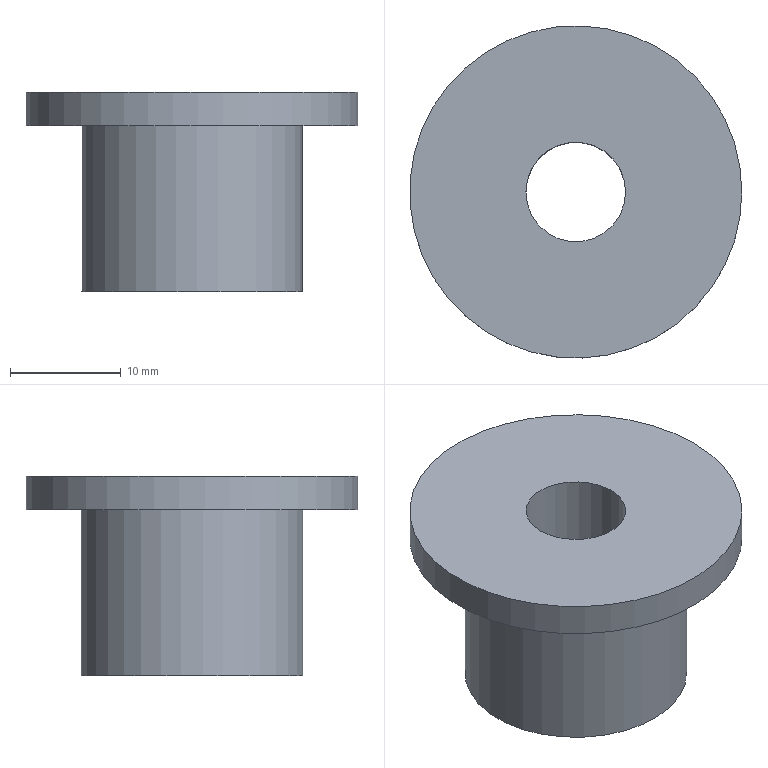Component | NX | ROLLING_SHAFT | 1 solid | 6 faces | box 30 x 30 x 18 mm | volume 5688 mm3 | cylinder 3 | plane 3 | commonest cylinder face diameters 30 x1 9 x1 20 x1
STEP:
#1=CARTESIAN_POINT('',(0.,0.,0.));
#2=DIRECTION('',(0.,0.,1.));
#3=DIRECTION('',(1.,0.,0.));
#4=AXIS2_PLACEMENT_3D('',#1,#2,#3);
#5=CARTESIAN_POINT('',(1475.132,1212.,819.574));
#6=VERTEX_POINT('',#5);
#7=CARTESIAN_POINT('',(1460.132,1212.,819.574));
#8=DIRECTION('',(0.,0.,1.));
#9=DIRECTION('',(1.,0.,0.));
#10=AXIS2_PLACEMENT_3D('',#7,#8,#9);
#11=CIRCLE('',#10,15.);
#12=CARTESIAN_POINT('',(1460.132,1212.,819.574));
#13=DIRECTION('',(0.,0.,1.));
#14=DIRECTION('',(1.,0.,0.));
#15=AXIS2_PLACEMENT_3D('',#12,#13,#14);
#16=CYLINDRICAL_SURFACE('',#15,15.);
#17=CARTESIAN_POINT('',(0.,0.));
#18=DIRECTION('',(1.,0.));
#19=VECTOR('',#18,1.);
#20=LINE('',#17,#19);
#21=(GEOMETRIC_REPRESENTATION_CONTEXT(2)PARAMETRIC_REPRESENTATION_CONTEXT()REPRESENTATION_CONTEXT('',''));
#22=DEFINITIONAL_REPRESENTATION('',(#20),#21);
#23=PCURVE('',#16,#22);
#24=CARTESIAN_POINT('',(1460.132,1212.,819.574));
#25=DIRECTION('',(0.,0.,1.));
#26=DIRECTION('',(1.,0.,0.));
#27=AXIS2_PLACEMENT_3D('',#24,#25,#26);
#28=PLANE('',#27);
#29=CARTESIAN_POINT('',(0.,0.));
#30=DIRECTION('',(1.,0.));
#31=AXIS2_PLACEMENT_2D('',#29,#30);
#32=CIRCLE('',#31,15.);
#33=(GEOMETRIC_REPRESENTATION_CONTEXT(2)PARAMETRIC_REPRESENTATION_CONTEXT()REPRESENTATION_CONTEXT('',''));
#34=DEFINITIONAL_REPRESENTATION('',(#32),#33);
#35=PCURVE('',#28,#34);
#36=SURFACE_CURVE('',#11,(#23,#35),.PCURVE_S1.);
#37=EDGE_CURVE('',#6,#6,#36,.T.);
#38=ORIENTED_EDGE('',*,*,#37,.T.);
#39=CARTESIAN_POINT('',(1475.132,1212.,822.574));
#40=VERTEX_POINT('',#39);
#41=CARTESIAN_POINT('',(1475.132,1212.,819.574));
#42=CARTESIAN_POINT('',(1475.132,1212.,822.574));
#43=B_SPLINE_CURVE_WITH_KNOTS('',1,(#41,#42),.UNSPECIFIED.,.F.,.F.,(2,2),(0.,3.),.PIECEWISE_BEZIER_KNOTS.);
#44=CARTESIAN_POINT('',(6.283,0.));
#45=DIRECTION('',(0.,1.));
#46=VECTOR('',#45,1.);
#47=LINE('',#44,#46);
#48=(GEOMETRIC_REPRESENTATION_CONTEXT(2)PARAMETRIC_REPRESENTATION_CONTEXT()REPRESENTATION_CONTEXT('',''));
#49=DEFINITIONAL_REPRESENTATION('',(#47),#48);
#50=PCURVE('',#16,#49);
#51=CARTESIAN_POINT('',(0.,0.));
#52=DIRECTION('',(0.,1.));
#53=VECTOR('',#52,1.);
#54=LINE('',#51,#53);
#55=(GEOMETRIC_REPRESENTATION_CONTEXT(2)PARAMETRIC_REPRESENTATION_CONTEXT()REPRESENTATION_CONTEXT('',''));
#56=DEFINITIONAL_REPRESENTATION('',(#54),#55);
#57=PCURVE('',#16,#56);
#58=SEAM_CURVE('',#43,(#50,#57),.PCURVE_S1.);
#59=EDGE_CURVE('',#6,#40,#58,.T.);
#60=ORIENTED_EDGE('',*,*,#59,.T.);
#61=CARTESIAN_POINT('',(1460.132,1212.,822.574));
#62=DIRECTION('',(0.,0.,1.));
#63=DIRECTION('',(1.,0.,0.));
#64=AXIS2_PLACEMENT_3D('',#61,#62,#63);
#65=CIRCLE('',#64,15.);
#66=CARTESIAN_POINT('',(0.,3.));
#67=DIRECTION('',(1.,0.));
#68=VECTOR('',#67,1.);
#69=LINE('',#66,#68);
#70=(GEOMETRIC_REPRESENTATION_CONTEXT(2)PARAMETRIC_REPRESENTATION_CONTEXT()REPRESENTATION_CONTEXT('',''));
#71=DEFINITIONAL_REPRESENTATION('',(#69),#70);
#72=PCURVE('',#16,#71);
#73=CARTESIAN_POINT('',(1460.132,1212.,822.574));
#74=DIRECTION('',(0.,0.,1.));
#75=DIRECTION('',(1.,0.,0.));
#76=AXIS2_PLACEMENT_3D('',#73,#74,#75);
#77=PLANE('',#76);
#78=CARTESIAN_POINT('',(0.,0.));
#79=DIRECTION('',(1.,0.));
#80=AXIS2_PLACEMENT_2D('',#78,#79);
#81=CIRCLE('',#80,15.);
#82=(GEOMETRIC_REPRESENTATION_CONTEXT(2)PARAMETRIC_REPRESENTATION_CONTEXT()REPRESENTATION_CONTEXT('',''));
#83=DEFINITIONAL_REPRESENTATION('',(#81),#82);
#84=PCURVE('',#77,#83);
#85=SURFACE_CURVE('',#65,(#72,#84),.PCURVE_S1.);
#86=EDGE_CURVE('',#40,#40,#85,.T.);
#87=ORIENTED_EDGE('',*,*,#86,.F.);
#88=ORIENTED_EDGE('',*,*,#59,.F.);
#89=EDGE_LOOP('',(#38,#60,#87,#88));
#90=FACE_BOUND('',#89,.T.);
#91=ADVANCED_FACE('',(#90),#16,.T.);
#92=CARTESIAN_POINT('',(1464.632,1212.,822.574));
#93=VERTEX_POINT('',#92);
#94=CARTESIAN_POINT('',(1460.132,1212.,822.574));
#95=DIRECTION('',(0.,0.,1.));
#96=DIRECTION('',(1.,0.,0.));
#97=AXIS2_PLACEMENT_3D('',#94,#95,#96);
#98=CIRCLE('',#97,4.5);
#99=CARTESIAN_POINT('',(1460.132,1212.,819.574));
#100=DIRECTION('',(0.,0.,1.));
#101=DIRECTION('',(1.,0.,0.));
#102=AXIS2_PLACEMENT_3D('',#99,#100,#101);
#103=CYLINDRICAL_SURFACE('',#102,4.5);
#104=CARTESIAN_POINT('',(0.,3.));
#105=DIRECTION('',(1.,0.));
#106=VECTOR('',#105,1.);
#107=LINE('',#104,#106);
#108=(GEOMETRIC_REPRESENTATION_CONTEXT(2)PARAMETRIC_REPRESENTATION_CONTEXT()REPRESENTATION_CONTEXT('',''));
#109=DEFINITIONAL_REPRESENTATION('',(#107),#108);
#110=PCURVE('',#103,#109);
#111=CARTESIAN_POINT('',(0.,0.));
#112=DIRECTION('',(1.,0.));
#113=AXIS2_PLACEMENT_2D('',#111,#112);
#114=CIRCLE('',#113,4.5);
#115=(GEOMETRIC_REPRESENTATION_CONTEXT(2)PARAMETRIC_REPRESENTATION_CONTEXT()REPRESENTATION_CONTEXT('',''));
#116=DEFINITIONAL_REPRESENTATION('',(#114),#115);
#117=PCURVE('',#77,#116);
#118=SURFACE_CURVE('',#98,(#110,#117),.PCURVE_S1.);
#119=EDGE_CURVE('',#93,#93,#118,.T.);
#120=ORIENTED_EDGE('',*,*,#119,.F.);
#121=CARTESIAN_POINT('',(1464.632,1212.,804.574));
#122=VERTEX_POINT('',#121);
#123=CARTESIAN_POINT('',(1464.632,1212.,804.574));
#124=CARTESIAN_POINT('',(1464.632,1212.,822.574));
#125=B_SPLINE_CURVE_WITH_KNOTS('',1,(#123,#124),.UNSPECIFIED.,.F.,.F.,(2,2),(-15.,3.),.PIECEWISE_BEZIER_KNOTS.);
#126=CARTESIAN_POINT('',(0.,0.));
#127=DIRECTION('',(0.,1.));
#128=VECTOR('',#127,1.);
#129=LINE('',#126,#128);
#130=(GEOMETRIC_REPRESENTATION_CONTEXT(2)PARAMETRIC_REPRESENTATION_CONTEXT()REPRESENTATION_CONTEXT('',''));
#131=DEFINITIONAL_REPRESENTATION('',(#129),#130);
#132=PCURVE('',#103,#131);
#133=CARTESIAN_POINT('',(6.283,0.));
#134=DIRECTION('',(0.,1.));
#135=VECTOR('',#134,1.);
#136=LINE('',#133,#135);
#137=(GEOMETRIC_REPRESENTATION_CONTEXT(2)PARAMETRIC_REPRESENTATION_CONTEXT()REPRESENTATION_CONTEXT('',''));
#138=DEFINITIONAL_REPRESENTATION('',(#136),#137);
#139=PCURVE('',#103,#138);
#140=SEAM_CURVE('',#125,(#132,#139),.PCURVE_S1.);
#141=EDGE_CURVE('',#122,#93,#140,.T.);
#142=ORIENTED_EDGE('',*,*,#141,.F.);
#143=CARTESIAN_POINT('',(1460.132,1212.,804.574));
#144=DIRECTION('',(0.,0.,-1.));
#145=DIRECTION('',(1.,0.,0.));
#146=AXIS2_PLACEMENT_3D('',#143,#144,#145);
#147=CIRCLE('',#146,4.5);
#148=CARTESIAN_POINT('',(6.283,-15.));
#149=DIRECTION('',(-1.,0.));
#150=VECTOR('',#149,1.);
#151=LINE('',#148,#150);
#152=(GEOMETRIC_REPRESENTATION_CONTEXT(2)PARAMETRIC_REPRESENTATION_CONTEXT()REPRESENTATION_CONTEXT('',''));
#153=DEFINITIONAL_REPRESENTATION('',(#151),#152);
#154=PCURVE('',#103,#153);
#155=CARTESIAN_POINT('',(1460.132,1212.,804.574));
#156=DIRECTION('',(0.,0.,-1.));
#157=DIRECTION('',(-1.,0.,0.));
#158=AXIS2_PLACEMENT_3D('',#155,#156,#157);
#159=PLANE('',#158);
#160=CARTESIAN_POINT('',(0.,0.));
#161=DIRECTION('',(-1.,0.));
#162=AXIS2_PLACEMENT_2D('',#160,#161);
#163=CIRCLE('',#162,4.5);
#164=(GEOMETRIC_REPRESENTATION_CONTEXT(2)PARAMETRIC_REPRESENTATION_CONTEXT()REPRESENTATION_CONTEXT('',''));
#165=DEFINITIONAL_REPRESENTATION('',(#163),#164);
#166=PCURVE('',#159,#165);
#167=SURFACE_CURVE('',#147,(#154,#166),.PCURVE_S1.);
#168=EDGE_CURVE('',#122,#122,#167,.T.);
#169=ORIENTED_EDGE('',*,*,#168,.F.);
#170=ORIENTED_EDGE('',*,*,#141,.T.);
#171=EDGE_LOOP('',(#120,#142,#169,#170));
#172=FACE_BOUND('',#171,.F.);
#173=ADVANCED_FACE('',(#172),#103,.F.);
#174=CARTESIAN_POINT('',(1470.132,1212.,819.574));
#175=VERTEX_POINT('',#174);
#176=CARTESIAN_POINT('',(1460.132,1212.,819.574));
#177=DIRECTION('',(0.,0.,-1.));
#178=DIRECTION('',(1.,0.,0.));
#179=AXIS2_PLACEMENT_3D('',#176,#177,#178);
#180=CIRCLE('',#179,10.);
#181=CARTESIAN_POINT('',(10.,0.));
#182=CARTESIAN_POINT('',(10.,-17.321));
#183=CARTESIAN_POINT('',(-5.,-8.66));
#184=CARTESIAN_POINT('',(-20.,-0.));
#185=CARTESIAN_POINT('',(-5.,8.66));
#186=CARTESIAN_POINT('',(10.,17.321));
#187=CARTESIAN_POINT('',(10.,0.));
#188=(BOUNDED_CURVE()B_SPLINE_CURVE(2,(#181,#182,#183,#184,#185,#186,#187),.UNSPECIFIED.,.T.,.F.)B_SPLINE_CURVE_WITH_KNOTS((1,2,2,2,2,1),(-2.094,0.,2.094,4.189,6.283,8.378),.UNSPECIFIED.)CURVE()GEOMETRIC_REPRESENTATION_ITEM()RATIONAL_B_SPLINE_CURVE((1.,0.5,1.,0.5,1.,0.5,1.))REPRESENTATION_ITEM(''));
#189=(GEOMETRIC_REPRESENTATION_CONTEXT(2)PARAMETRIC_REPRESENTATION_CONTEXT()REPRESENTATION_CONTEXT('',''));
#190=DEFINITIONAL_REPRESENTATION('',(#188),#189);
#191=PCURVE('',#28,#190);
#192=CARTESIAN_POINT('',(1460.132,1212.,804.574));
#193=DIRECTION('',(0.,0.,1.));
#194=DIRECTION('',(1.,0.,0.));
#195=AXIS2_PLACEMENT_3D('',#192,#193,#194);
#196=CYLINDRICAL_SURFACE('',#195,10.);
#197=CARTESIAN_POINT('',(6.283,15.));
#198=DIRECTION('',(-1.,0.));
#199=VECTOR('',#198,1.);
#200=LINE('',#197,#199);
#201=(GEOMETRIC_REPRESENTATION_CONTEXT(2)PARAMETRIC_REPRESENTATION_CONTEXT()REPRESENTATION_CONTEXT('',''));
#202=DEFINITIONAL_REPRESENTATION('',(#200),#201);
#203=PCURVE('',#196,#202);
#204=SURFACE_CURVE('',#180,(#191,#203),.PCURVE_S1.);
#205=EDGE_CURVE('',#175,#175,#204,.T.);
#206=ORIENTED_EDGE('',*,*,#205,.F.);
#207=EDGE_LOOP('',(#206));
#208=FACE_BOUND('',#207,.T.);
#209=ORIENTED_EDGE('',*,*,#37,.F.);
#210=EDGE_LOOP('',(#209));
#211=FACE_BOUND('',#210,.T.);
#212=ADVANCED_FACE('',(#208,#211),#28,.F.);
#213=ORIENTED_EDGE('',*,*,#86,.T.);
#214=EDGE_LOOP('',(#213));
#215=FACE_BOUND('',#214,.T.);
#216=ORIENTED_EDGE('',*,*,#119,.F.);
#217=EDGE_LOOP('',(#216));
#218=FACE_BOUND('',#217,.T.);
#219=ADVANCED_FACE('',(#215,#218),#77,.T.);
#220=CARTESIAN_POINT('',(1470.132,1212.,804.574));
#221=VERTEX_POINT('',#220);
#222=CARTESIAN_POINT('',(1460.132,1212.,804.574));
#223=DIRECTION('',(0.,0.,-1.));
#224=DIRECTION('',(1.,0.,0.));
#225=AXIS2_PLACEMENT_3D('',#222,#223,#224);
#226=CIRCLE('',#225,10.);
#227=CARTESIAN_POINT('',(6.283,0.));
#228=DIRECTION('',(-1.,0.));
#229=VECTOR('',#228,1.);
#230=LINE('',#227,#229);
#231=(GEOMETRIC_REPRESENTATION_CONTEXT(2)PARAMETRIC_REPRESENTATION_CONTEXT()REPRESENTATION_CONTEXT('',''));
#232=DEFINITIONAL_REPRESENTATION('',(#230),#231);
#233=PCURVE('',#196,#232);
#234=CARTESIAN_POINT('',(0.,0.));
#235=DIRECTION('',(-1.,0.));
#236=AXIS2_PLACEMENT_2D('',#234,#235);
#237=CIRCLE('',#236,10.);
#238=(GEOMETRIC_REPRESENTATION_CONTEXT(2)PARAMETRIC_REPRESENTATION_CONTEXT()REPRESENTATION_CONTEXT('',''));
#239=DEFINITIONAL_REPRESENTATION('',(#237),#238);
#240=PCURVE('',#159,#239);
#241=SURFACE_CURVE('',#226,(#233,#240),.PCURVE_S1.);
#242=EDGE_CURVE('',#221,#221,#241,.T.);
#243=ORIENTED_EDGE('',*,*,#242,.F.);
#244=CARTESIAN_POINT('',(1470.132,1212.,804.574));
#245=CARTESIAN_POINT('',(1470.132,1212.,819.574));
#246=B_SPLINE_CURVE_WITH_KNOTS('',1,(#244,#245),.UNSPECIFIED.,.F.,.F.,(2,2),(0.,15.),.PIECEWISE_BEZIER_KNOTS.);
#247=CARTESIAN_POINT('',(6.283,0.));
#248=DIRECTION('',(0.,1.));
#249=VECTOR('',#248,1.);
#250=LINE('',#247,#249);
#251=(GEOMETRIC_REPRESENTATION_CONTEXT(2)PARAMETRIC_REPRESENTATION_CONTEXT()REPRESENTATION_CONTEXT('',''));
#252=DEFINITIONAL_REPRESENTATION('',(#250),#251);
#253=PCURVE('',#196,#252);
#254=CARTESIAN_POINT('',(0.,0.));
#255=DIRECTION('',(0.,1.));
#256=VECTOR('',#255,1.);
#257=LINE('',#254,#256);
#258=(GEOMETRIC_REPRESENTATION_CONTEXT(2)PARAMETRIC_REPRESENTATION_CONTEXT()REPRESENTATION_CONTEXT('',''));
#259=DEFINITIONAL_REPRESENTATION('',(#257),#258);
#260=PCURVE('',#196,#259);
#261=SEAM_CURVE('',#246,(#253,#260),.PCURVE_S1.);
#262=EDGE_CURVE('',#221,#175,#261,.T.);
#263=ORIENTED_EDGE('',*,*,#262,.T.);
#264=ORIENTED_EDGE('',*,*,#205,.T.);
#265=ORIENTED_EDGE('',*,*,#262,.F.);
#266=EDGE_LOOP('',(#243,#263,#264,#265));
#267=FACE_BOUND('',#266,.T.);
#268=ADVANCED_FACE('',(#267),#196,.T.);
#269=ORIENTED_EDGE('',*,*,#242,.T.);
#270=EDGE_LOOP('',(#269));
#271=FACE_BOUND('',#270,.T.);
#272=ORIENTED_EDGE('',*,*,#168,.F.);
#273=EDGE_LOOP('',(#272));
#274=FACE_BOUND('',#273,.T.);
#275=ADVANCED_FACE('',(#271,#274),#159,.T.);
#276=CLOSED_SHELL('',(#91,#173,#212,#219,#268,#275));
#277=MANIFOLD_SOLID_BREP('',#276);
#278=(LENGTH_UNIT()NAMED_UNIT(*)SI_UNIT(.MILLI.,.METRE.));
#279=UNCERTAINTY_MEASURE_WITH_UNIT(LENGTH_MEASURE(0.00001),#278,'','');
#280=(NAMED_UNIT(*)PLANE_ANGLE_UNIT()SI_UNIT($,.RADIAN.));
#281=(NAMED_UNIT(*)SI_UNIT($,.STERADIAN.)SOLID_ANGLE_UNIT());
#282=(GEOMETRIC_REPRESENTATION_CONTEXT(3)GLOBAL_UNCERTAINTY_ASSIGNED_CONTEXT((#279))GLOBAL_UNIT_ASSIGNED_CONTEXT((#278,#280,#281))REPRESENTATION_CONTEXT('',''));
#283=ADVANCED_BREP_SHAPE_REPRESENTATION('',(#4,#277),#282);